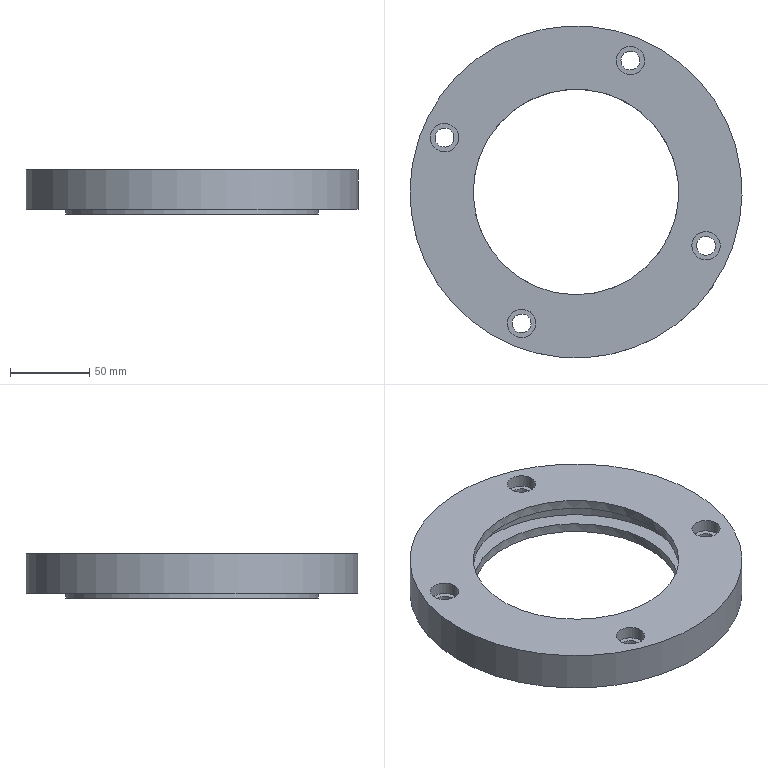Component | NX | CA6140-ZHUZHOU-DUANGAIYOU | 2 solids | 26 faces | volume 468364 mm3 | cylinder 15 | plane 11 | commonest cylinder face diameters 18 x4 12 x4 150 x3 130 x2 160 x1 210 x1